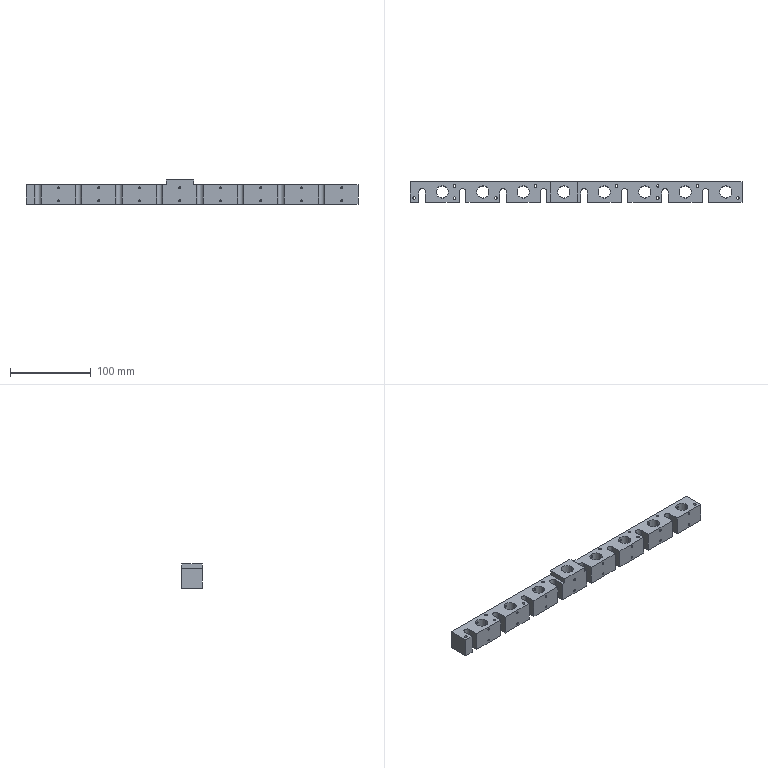Component | SolidWorks | 002MaterialPickingModuleB-1_004SidePlugModuleB-1_J-026-2 | 1 solid | 174 faces | box 410 x 25 x 30 mm | volume 188018 mm3 | cylinder 128 | plane 42 | cone 4 | commonest cylinder face diameters 2.5 x64 6.5 x16 3.4 x16 15 x16 8.1 x8 3 x4 3.3 x4 | material 45
build123d program:
from build123d import *

# Parameters (mm, degrees)
SKETCH1_W                                       = 440
SKETCH1_H                                       = 24
BOSS_EXTRUDE1_DEPTH                             = 12.5
SKETCH2_R                                       = 7.5
CUT_EXTRUDE1_DEPTH                              = 222.658
CUT_EXTRUDE2_DEPTH                              = 222.658
LPATTERN1_COUNT                                 = 8
LPATTERN1_PITCH                                 = 50
SKETCH4_W                                       = 34
SKETCH4_H                                       = 25
SKETCH4_R                                       = 7.5
BOSS_EXTRUDE2_DEPTH                             = 6
M4_TAPPED_HOLE1_D                               = 3.3
M4_TAPPED_HOLE1_DEPTH                           = 10.1
M4_TAPPED_HOLE1_TIP                             = 0.9914
SKETCH8_W                                       = 30
SKETCH8_H                                       = 25
CUT_EXTRUDE4_DEPTH                              = 223.388
M3_HEX_SOCKET_HEAD_CAP_SCREW_CBORE1_D           = 3.4
M3_HEX_SOCKET_HEAD_CAP_SCREW_CBORE1_CBORE_D     = 6.5
M3_HEX_SOCKET_HEAD_CAP_SCREW_CBORE1_CBORE_DEPTH = 3.4
SIZE_MM_DOWEL_PIN_HOLE1_D                       = 3
M3_TAPPED_HOLE1_D                               = 2.5
LPATTERN2_COUNT                                 = 8
LPATTERN2_PITCH                                 = 50


with BuildPart() as part:
    # Sketch1 → Boss-Extrude1 (new, symmetric)
    with BuildSketch(Plane(origin=(0, 0, 0), x_dir=(1, 0, 0), z_dir=(0, 1, 0))):
        Rectangle(SKETCH1_W, SKETCH1_H)
    extrude(amount=BOSS_EXTRUDE1_DEPTH, both=True)

    # Sketch2 → Cut-Extrude1 (cut, through all)
    with BuildSketch(Plane.XY.offset(12)):
        Circle(SKETCH2_R)
        with Locations((-50, 0)):
            Circle(SKETCH2_R)
        with Locations((-100, 0)):
            Circle(SKETCH2_R)
        with Locations((50, 0)):
            Circle(SKETCH2_R)
        with Locations((100, 0)):
            Circle(SKETCH2_R)
        with Locations((-150, 0)):
            Circle(SKETCH2_R)
        with Locations((150, 0)):
            Circle(SKETCH2_R)
        with Locations((-200, 0)):
            Circle(SKETCH2_R)
        with Locations((200, 0)):
            Circle(SKETCH2_R)
    extrude(amount=-CUT_EXTRUDE1_DEPTH, mode=Mode.SUBTRACT)

    # Sketch3 → Cut-Extrude2 (cut, through all)
    with BuildSketch(Plane.XY.offset(12)):
        with BuildLine():
            Line((-170.95, 0), (-170.95, -12.5))
            ThreePointArc((-170.95, -12.5), (-175, -16.55), (-179.05, -12.5))
            Line((-179.05, -12.5), (-179.05, 0))
            ThreePointArc((-179.05, 0), (-175, 4.05), (-170.95, 0))
        make_face()
    cut_extrude2 = extrude(amount=-CUT_EXTRUDE2_DEPTH, mode=Mode.SUBTRACT)

    # LPattern1: Cut-Extrude2 ×8
    with Locations(*[(i * LPATTERN1_PITCH, 0, 0) for i in range(1, LPATTERN1_COUNT)]):
        add(cut_extrude2, mode=Mode.SUBTRACT)

    # Sketch4 → Boss-Extrude2 (add)
    with BuildSketch(Plane(origin=(0, 0, -12), x_dir=(-1, 0, 0), z_dir=(0, 0, -1))):
        Rectangle(SKETCH4_W, SKETCH4_H)
        with Locations(Location((0, 0, 0), (0, 0, 180))):
            Circle(SKETCH4_R, mode=Mode.SUBTRACT)
    extrude(amount=BOSS_EXTRUDE2_DEPTH)

    # M4 Tapped Hole1
    with Locations(Plane(origin=(0, 12.5, 0), x_dir=(1, 0, 0), z_dir=(0, 1, 0))):
        with Locations((12.5, 13), (12.5, -6)):
            Hole(M4_TAPPED_HOLE1_D / 2, depth=M4_TAPPED_HOLE1_DEPTH)
            with Locations((0, 0, -(M4_TAPPED_HOLE1_DEPTH + M4_TAPPED_HOLE1_TIP / 2))):  # 118° drill point
                Cone(0, M4_TAPPED_HOLE1_D / 2, M4_TAPPED_HOLE1_TIP, mode=Mode.SUBTRACT)

    # Sketch8 → Cut-Extrude4 (cut, through all)
    with BuildSketch(Plane.XY.offset(12)):
        with Locations((205, 0)):
            Rectangle(SKETCH8_W, SKETCH8_H)
    extrude(amount=-CUT_EXTRUDE4_DEPTH, mode=Mode.SUBTRACT)

    # M3 Hex Socket Head Cap Screw CBORE1 (through all)
    with Locations(Plane.XY.offset(12)):
        with Locations((-215, -7.5), (-165, 7.5), (-115.95, -7.5), (-65, 7.5), (35, 7.5), (84.05, -7.5), (135, 7.5), (185, -7.5)):
            CounterBoreHole(M3_HEX_SOCKET_HEAD_CAP_SCREW_CBORE1_D / 2, M3_HEX_SOCKET_HEAD_CAP_SCREW_CBORE1_CBORE_D / 2, M3_HEX_SOCKET_HEAD_CAP_SCREW_CBORE1_CBORE_DEPTH)

    # Size mm Dowel Pin Hole1 (through all)
    with Locations(Plane.XY.offset(12)):
        with Locations((-115.95, 7.5), (135, -7.5)):
            Hole(SIZE_MM_DOWEL_PIN_HOLE1_D / 2)

    # M3 Tapped Hole1 (through all)
    with Locations(Plane(origin=(0, 12.5, 0), x_dir=(1, 0, 0), z_dir=(0, 1, 0))):
        with Locations((150, -8), (150, 8)):
            m3_tapped_hole1 = Hole(M3_TAPPED_HOLE1_D / 2)

    # LPattern2: M3 Tapped Hole1 ×8
    with Locations(*[(-i * LPATTERN2_PITCH, 0, 0) for i in range(1, LPATTERN2_COUNT)]):
        add(m3_tapped_hole1, mode=Mode.SUBTRACT)


solid = part.part

# Placed as in the assembly
solid = solid.moved(Location((220.326, 296.019, 101.231), (-180, 0, 180)))